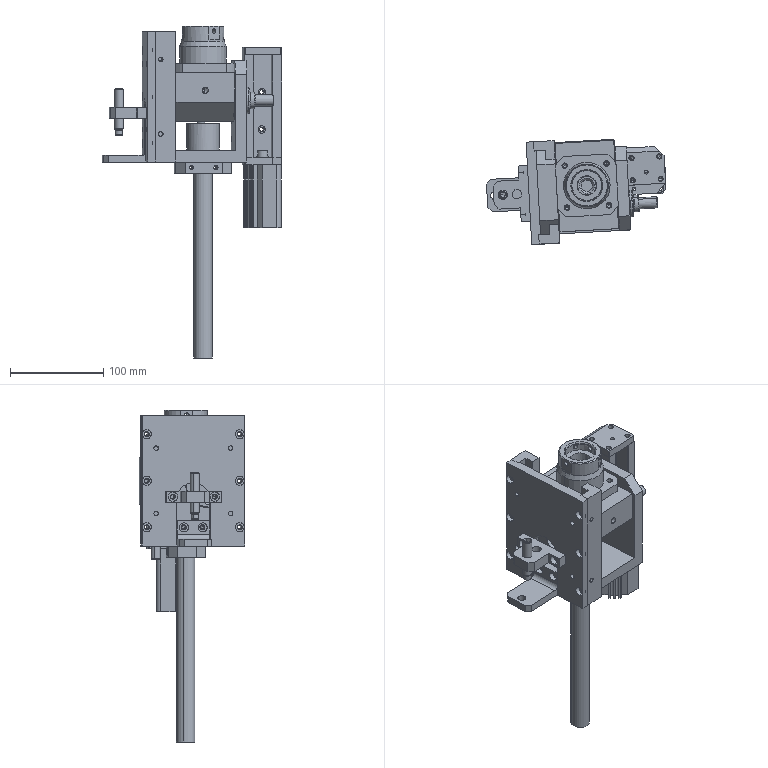Assembly | SolidWorks | mm | 23 component files | 23 solids | 814 faces | box 192.24 x 112.98 x 356.4 mm | volume 1271126 mm3 | cylinder 366 | plane 316 | cone 106 | torus 26 | commonest cylinder face diameters 4.2 x58 5.5 x44 5 x30 10 x27 8 x24 9 x16 9.8 x12 4.26 x10
Bill of materials:
BearingPressPartG | 1 |  | Flat rectangular plate with a U-shaped slot (round-ended) open at one edge, a stepped/rebated strip along one long side, and a symmetric pattern of small through holes.
BearingPressPartH | 2 |  | Long prismatic bar with an L-shaped (stepped) cross-section and a row of three through holes along one face.
BearingPressPartI | 1 |  | Thick L-shaped angle bracket with an inside fillet; one leg has a single through hole, the other leg has two through holes; outer corners of the single-hole leg are chamfered.
BearingPressPartK | 1 |  | T-shaped block: a long rectangular bar with two cross holes through its side faces, joined to a chamfered tab carrying two vertical through holes.
BearingPressPartL | 1 |  | Thick-walled cylindrical sleeve with a coaxial bore; one end has a reduced-diameter portion cut into two opposed tabs separated by a slot, each tab carrying a small cross hole.
BearingPressPartM | 1 |  | Octagonal (chamfered-rectangle) thick plate with a large central cutout combining a circle with a wider flat-ended slot, two vertical through holes at the ends, and horizontal holes through the long side faces into the cutout.
BearingPressPartN | 1 |  | Long, slender thin-walled circular tube with plain ends.
BearingPressPartPLeft | 1 |  | U-shaped bracket with two parallel upright side plates joined by a base plate; side plates have chamfered top corners, a large central hole with a shallow circular counterbore/recess, small holes around it, and a column of holes near one edge; base has a large hole and smaller holes.
BearingPressPartQ | 1 |  | Rectangular block with a large stepped bore through the top face surrounded by four small holes, a keyed bore through one side face, a smaller cross hole, and a chamfered lower corner on one end.
MPSZ18-20 | 2 | Tin Bronze | Thin circular flange plate with a cylindrical hub on one side. A large central bore goes through the hub, and two countersunk holes sit diametrically opposite each other on the flange.
MSSG10-50 | 2 | S45C | Solid stepped cylindrical pin: a long main body plus a short, smaller-diameter coaxial end section. Both ends are chamfered.
STEHN14 | 1 | SUJ2 | Hex-headed part with a short, plain cylindrical shank. The shank has a chamfered free end and a slightly smaller neck/undercut next to the head.
T160418-M01U03-P04A | 1 | Tin Bronze | Long prismatic column with a C/U-shaped channel cross-section (with small internal steps) running the full length, four axial holes in the end face, and two transverse holes on one side face.
T160418-M01U03-P08 | 1 | SKS3 | Flanged cylindrical housing: square flange with chamfered corners and four holes, a stepped cylindrical body with a central through bore and internal counterbore, and radial holes near the upper end with local flats.
T160418-M01U03-P09 | 1 | SCr440 | Headed stepped pin/shaft: a thin round head, long main cylindrical shank, a short groove, and a reduced-diameter end journal with a small axial center hole.
T160418-M01U03-P10 | 1 | S45C | Flat annular ring (washer-like) with a large concentric through bore, a rectangular cross-section, and slightly rounded outer edges.
T160418-M01U03-P11A | 1 | S45C | Thick, roughly square flat plate with four through holes near the corners and one smaller central through hole. One corner has a large angled chamfer; the other corners have small corner breaks.
T160418-M01U03-P13A | 1 | S45C | Flat, irregular polygonal plate with one large round through hole and six smaller round through holes around it. It has two large angled chamfers on adjacent corners and small breaks on the remaining corners.
Mates:
1. coincident | BearingPressPartG-1 face at (391.069, 164.922, -283.818) dir (0.9985, 0.05472, 0) | BearingPressPartH-1 face at (391.069, 164.922, -143.818) dir (-0.9985, -0.05472, 0)
2. coincident | BearingPressPartG-1 face at (390.522, 174.907, -283.818) dir (-0.05472, 0.9985, 0) | BearingPressPartH-1 face at (412.489, 176.111, -143.818) dir (-0.05472, 0.9985, 0)
3. concentric | BearingPressPartG-1 face at (382.808, 169.477, -163.818) dir (-0.9985, -0.05472, 0) r 4.9 | BearingPressPartH-1 face at (412.763, 171.118, -163.818) dir (0.9985, 0.05472, 0) r 2.1
4. coincident | BearingPressPartG-1 face at (396.541, 65.072, -283.818) dir (0.9985, 0.05472, 0) | BearingPressPartH-2 face at (395.994, 75.057, -283.818) dir (-0.9985, -0.05472, 0)
5. coincident | BearingPressPartH-1 face at (403.598, 155.593, -283.818) dir (0, 0, -1) | BearingPressPartH-2 face at (407.429, 85.698, -283.818) dir (0, 0, -1)
6. coincident | BearingPressPartG-1 face at (388.553, 64.634, -283.818) dir (0.05472, -0.9985, 0) | BearingPressPartH-2 face at (418.508, 66.275, -283.818) dir (0.05472, -0.9985, 0)
7. coincident | T160418-M01U03-P04A-1 face at (492.226, 128.272, -168.818) dir (0, 0, 1) | T160418-M01U03-P11A-1 face at (492.226, 128.272, -168.818) dir (0, 0, -1)
8. concentric | T160418-M01U03-P04A-1 face at (525.587, 159.144, -168.818) dir (0, 0, 1) r 2.1 | T160418-M01U03-P11A-1 face at (525.587, 159.144, -168.818) dir (0, 0, -1) r 2.75
9. concentric | T160418-M01U03-P04A-1 face at (495.632, 157.502, -168.818) dir (0, 0, 1) r 2.1 | T160418-M01U03-P11A-1 face at (495.632, 157.502, -168.818) dir (0, 0, -1) r 2.75
10. concentric | T160418-M01U03-P04A-1 face at (495.632, 157.502, -278.818) dir (0, 0, -1) r 2.1 | T160418-M01U03-P13A-1 face at (495.632, 157.502, -286.818) dir (0, 0, -1) r 4.5
11. concentric | T160418-M01U03-P04A-1 face at (515.602, 158.596, -278.818) dir (0, 0, -1) r 2.1 | T160418-M01U03-P13A-1 face at (515.602, 158.596, -286.818) dir (0, 0, -1) r 4.5
12. coincident | T160418-M01U03-P04A-1 face at (492.226, 128.272, -278.818) dir (0, 0, -1) | T160418-M01U03-P13A-1 face at (490.038, 168.212, -278.818) dir (0, 0, 1)
13. coincident | T160418-M01U03-P13A-1 face at (490.038, 168.212, -286.818) dir (0, 0, -1) | CDQ2B25-35DZ-M9BL-1/CDQ2B25-35-M9B(0_0)_BODY-1 face at (525.791, 125.209, -286.818) dir (0, 0, 1)
14. concentric | T160418-M01U03-P13A-1 face at (511.649, 139.351, -278.818) dir (0, 0, -1) r 10 | CDQ2B25-35DZ-M9BL-1/CDQ2B25-35-M9B(0_0)_BODY-1 face at (511.649, 139.351, -354.318) dir (0, 0, -1) r 13
15. concentric | BearingPressPartG-1 face at (384.312, 142.018, -230.818) dir (-0.9985, -0.05472, 0) r 2.1 | BearingPressPartK-1 face at (374.327, 141.471, -230.818) dir (-0.9985, -0.05472, 0) r 5
16. coincident | BearingPressPartG-1 face at (382.534, 174.469, -283.818) dir (-0.9985, -0.05472, 0) | BearingPressPartK-1 face at (386.364, 104.574, -224.818) dir (0.9985, 0.05472, 0)
17. concentric | BearingPressPartG-1 face at (386.775, 97.085, -230.818) dir (-0.9985, -0.05472, 0) r 2.1 | BearingPressPartK-1 face at (376.79, 96.538, -230.818) dir (-0.9985, -0.05472, 0) r 5
18. concentric | BearingPressPartM-1 face at (447.676, 127.964, -295.818) dir (0, 0, 1) r 10.025 | BearingPressPartL-1 face at (447.676, 127.964, -242.818) dir (0, 0, -1) r 17.5
19. coincident | BearingPressPartM-1 face at (476.537, 149.575, -283.818) dir (0, 0, 1) | BearingPressPartL-1 face at (447.676, 127.964, -283.818) dir (0, 0, -1)
20. coincident | BearingPressPartM-1 face at (453.908, 135.817, -295.818) dir (0.05472, -0.9985, 0) | BearingPressPartL-1 face at (480.097, 137.252, -283.818) dir (-0.05472, 0.9985, 0)
21. coincident | STEHN14-1 face at (445.925, 159.916, -248.13) dir (0, 0, -1) | MSSG10-50-2 face at (444.73, 156.627, -248.13) dir (0, 0, 1)
22. coincident | BearingPressPartG-1 face at (397.991, 75.166, -283.818) dir (0.9985, 0.05472, 0) | BearingPressPartPLeft-1 face at (393.066, 165.031, -283.818) dir (-0.9985, -0.05472, 0)
23. width | BearingPressPartPLeft-1 face at (393.066, 165.031, -283.818) dir (-0.05472, 0.9985, 0) | BearingPressPartPLeft-1 face at (397.991, 75.166, -283.818) dir (0.05472, -0.9985, 0) | BearingPressPartH-2 face at (418.508, 66.275, -283.818) dir (0.05472, -0.9985, 0) | BearingPressPartH-1 face at (412.489, 176.111, -143.818) dir (-0.05472, 0.9985, 0)
24. coincident | BearingPressPartG-1 face at (388.553, 64.634, -283.818) dir (0, 0, -1) | BearingPressPartPLeft-1 face at (393.066, 165.031, -283.818) dir (0, 0, -1)
25. concentric | BearingPressPartL-1 face at (447.676, 127.964, -242.818) dir (0, 0, -1) r 17.5 | BearingPressPartPLeft-1 face at (447.676, 127.964, -283.818) dir (0, 0, 1) r 17.5
26. coincident | BearingPressPartM-1 face at (476.537, 149.575, -283.818) dir (0, 0, 1) | BearingPressPartPLeft-1 face at (393.066, 165.031, -283.818) dir (0, 0, -1)
27. coincident | BearingPressPartI-2 face at (394.571, 137.572, -284.318) dir (0.9985, 0.05472, 0) | BearingPressPartPLeft-1 face at (393.066, 165.031, -283.818) dir (-0.9985, -0.05472, 0)
28. concentric | BearingPressPartI-2 face at (388.088, 109.676, -263.818) dir (-0.9985, -0.05472, 0) r 5 | BearingPressPartPLeft-1 face at (396.076, 110.114, -263.818) dir (-0.9985, -0.05472, 0) r 2.1
29. concentric | BearingPressPartK-1 face at (357.585, 118.019, -224.818) dir (0, 0, 1) r 5 | MSSG10-50-3 face at (357.585, 118.019, -255.241) dir (0, 0, 1) r 5
30. concentric | MSSG10-50-2 face at (445.925, 159.916, -248.13) dir (0, 0, -1) r 5 | BearingPressPartPLeft-1 face at (445.925, 159.916, -271.818) dir (0, 0, 1) r 5
31. concentric | STEHN14-1 face at (445.925, 159.916, -233.13) dir (0, 0, -1) r 4 | MSSG10-50-2 face at (445.925, 159.916, -248.13) dir (0, 0, -1) r 4
32. concentric | T160418-M01U03-P04A-1 face at (490.639, 157.228, -238.818) dir (-0.9985, -0.05472, 0) r 4 | BearingPressPartPLeft-1 face at (490.639, 157.228, -238.818) dir (0.9985, 0.05472, 0) r 4
33. concentric | T160418-M01U03-P04A-1 face at (490.639, 157.228, -218.818) dir (-0.9985, -0.05472, 0) r 4 | BearingPressPartPLeft-1 face at (490.639, 157.228, -218.818) dir (0.9985, 0.05472, 0) r 4
34. concentric | T160418-M01U03-P08-1 face at (447.676, 127.964, -167.818) dir (0, 0, -1) r 25 | BearingPressPartQ-1 face at (447.676, 127.964, -203.818) dir (0, 0, 1) r 18
35. concentric | T160418-M01U03-P08-1 face at (468.911, 151.661, -177.818) dir (0, 0, 1) r 3 | BearingPressPartQ-1 face at (468.911, 151.661, -187.818) dir (0, 0, 1) r 2.1
36. coincident | T160418-M01U03-P08-1 face at (447.676, 127.964, -187.818) dir (0, 0, -1) | BearingPressPartQ-1 face at (477.501, 177.67, -187.818) dir (0, 0, 1)
37. width | BearingPressPartPLeft-1 face at (413.036, 166.126, -271.818) dir (0.9985, 0.05472, 0) | BearingPressPartPLeft-1 face at (477.939, 169.682, -174.818) dir (-0.9985, -0.05472, 0) | BearingPressPartQ-1 face at (412.599, 174.114, -239.818) dir (-0.9985, -0.05472, 0) | BearingPressPartQ-1 face at (477.501, 177.67, -239.818) dir (0.9985, 0.05472, 0)
38. concentric | BearingPressPartPLeft-1 face at (396.459, 103.124, -217.818) dir (0.9985, 0.05472, 0) r 12 | BearingPressPartQ-1 face at (416.429, 104.218, -217.818) dir (0.9985, 0.05472, 0) r 9
39. coincident | T160418-M01U03-P04A-1 face at (490.038, 168.212, -278.818) dir (-0.9985, -0.05472, 0) | BearingPressPartPLeft-1 face at (489.921, 170.339, -283.818) dir (0.9985, 0.05472, 0)
40. concentric | BearingPressPartM-1 face at (471.64, 129.277, -295.818) dir (0, 0, -1) r 2.75 | BearingPressPartPLeft-1 face at (471.64, 129.277, -283.818) dir (0, 0, -1) r 2.1
41. angle | BearingPressPartQ-1 face at (477.501, 177.67, -239.818) dir (-0.05472, 0.9985, 0) | BearingPressPartH-1 face at (412.489, 176.111, -143.818) dir (-0.05472, 0.9985, 0)
42. coincident | BearingPressPartPLeft-1 face at (490.318, 108.268, -217.818) dir (0.9985, 0.05472, 0) | MPSZ18-20-1 face at (490.318, 108.268, -230.218) dir (-0.9985, -0.05472, 0)
43. concentric | BearingPressPartPLeft-1 face at (396.459, 103.124, -217.818) dir (0.9985, 0.05472, 0) r 12 | MPSZ18-20-1 face at (473.343, 107.337, -217.818) dir (0.9985, 0.05472, 0) r 12
44. concentric | BearingPressPartPLeft-1 face at (490.318, 108.268, -200.318) dir (0.9985, 0.05472, 0) r 1.25 | MPSZ18-20-1 face at (490.318, 108.268, -200.318) dir (0.9985, 0.05472, 0) r 1.75
45. concentric | BearingPressPartPLeft-1 face at (404.746, 103.578, -217.818) dir (-0.9985, -0.05472, 0) r 25 | MPSZ18-20-2 face at (421.721, 104.508, -217.818) dir (-0.9985, -0.05472, 0) r 12
46. coincident | BearingPressPartPLeft-1 face at (404.746, 103.578, -217.818) dir (-0.9985, -0.05472, 0) | MPSZ18-20-2 face at (404.746, 103.578, -230.218) dir (0.9985, 0.05472, 0)
47. concentric | BearingPressPartPLeft-1 face at (490.318, 108.268, -200.318) dir (0.9985, 0.05472, 0) r 1.25 | MPSZ18-20-2 face at (404.746, 103.578, -200.318) dir (-0.9985, -0.05472, 0) r 1.75
48. concentric | MPSZ18-20-2 face at (421.721, 104.508, -217.818) dir (-0.9985, -0.05472, 0) r 9 | T160418-M01U03-P09-1 face at (503.348, 108.982, -217.818) dir (-0.9985, -0.05472, 0) r 9
49. coincident | MPSZ18-20-2 face at (401.751, 103.414, -241.818) dir (-0.9985, -0.05472, 0) | T160418-M01U03-P09-1 face at (401.751, 103.414, -217.818) dir (0.9985, 0.05472, 0)
50. concentric | T160418-M01U03-P09-1 face at (503.348, 108.982, -217.818) dir (-0.9985, -0.05472, 0) r 9 | T160418-M01U03-P10-1 face at (493.313, 108.432, -217.818) dir (0.9985, 0.05472, 0) r 9.1
51. coincident | MPSZ18-20-1 face at (493.313, 108.432, -241.818) dir (0.9985, 0.05472, 0) | T160418-M01U03-P10-1 face at (493.313, 108.432, -217.818) dir (-0.9985, -0.05472, 0)
52. concentric | BearingPressPartL-1 face at (447.676, 127.964, -242.818) dir (0, 0, -1) r 10 | BearingPressPartN-1 face at (447.676, 127.964, -494.218) dir (0, 0, 1) r 10
53. distance | CDQ2B25-35M9B(0_0)_CYROD-1 face at (-10, 3, 0) dir (-1, 0, 0) | CDQ2B25-35-M9B(0_0)_BODY-1 face at (0, -14.142, 14.142) dir (-1, 0, 0)
54. concentric | CDQ2B25-35-M9B(0_0)_BODY-1 face at (50, 0, 0) dir (-1, 0, 0) r 6 | CDQ2B25-35M9B(0_0)_CYROD-1 face at (45, 0, 0) dir (-1, 0, 0) r 6
55. parallel | CDQ2B25-35-M9B(0_0)_BODY-1 face at (67.5, 8.284, 20) dir (0, 0, 1) | CDQ2B25-35M9B(0_0)_CYROD-1 face at (-5, -12, 5) dir (0, 0, 1)